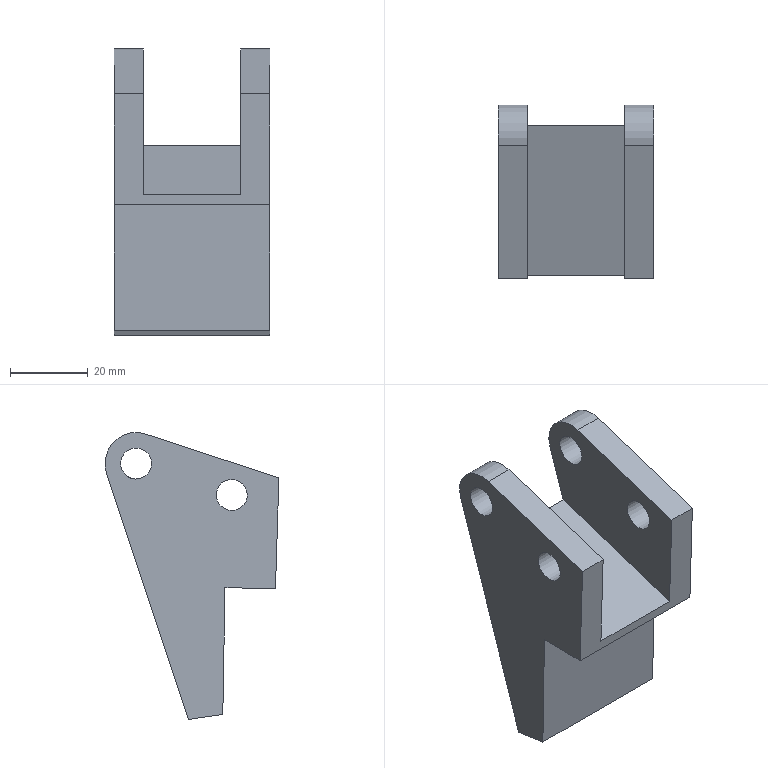Component | NX | JAW | 1 solid | 18 faces | volume 46721 mm3 | plane 12 | cylinder 6 | commonest cylinder face diameters 8 x4 16 x2